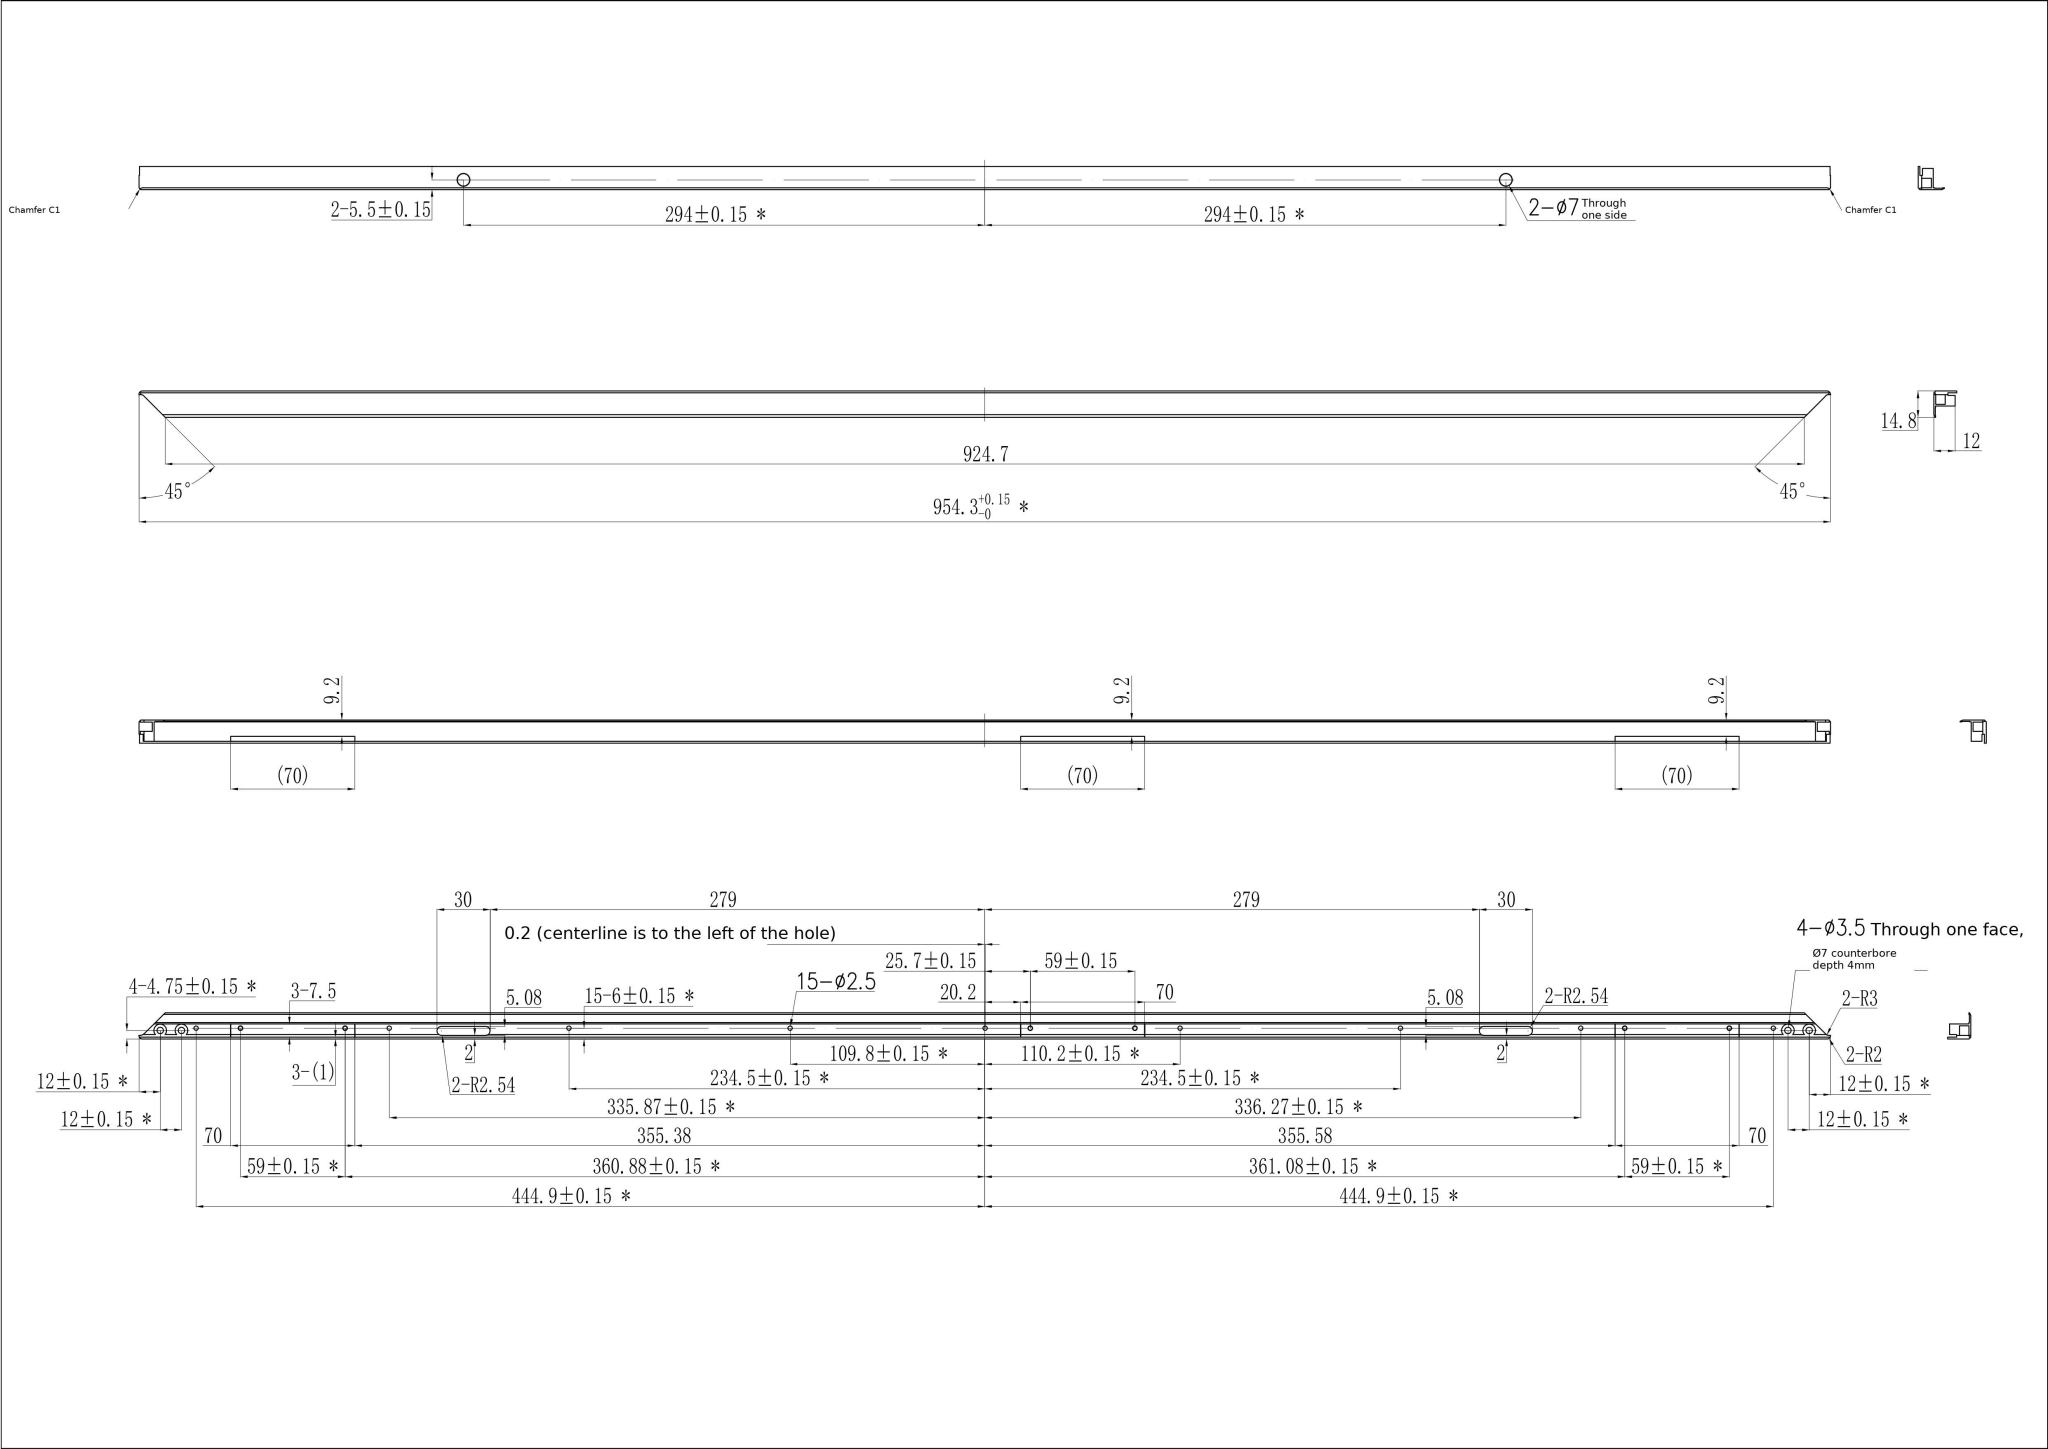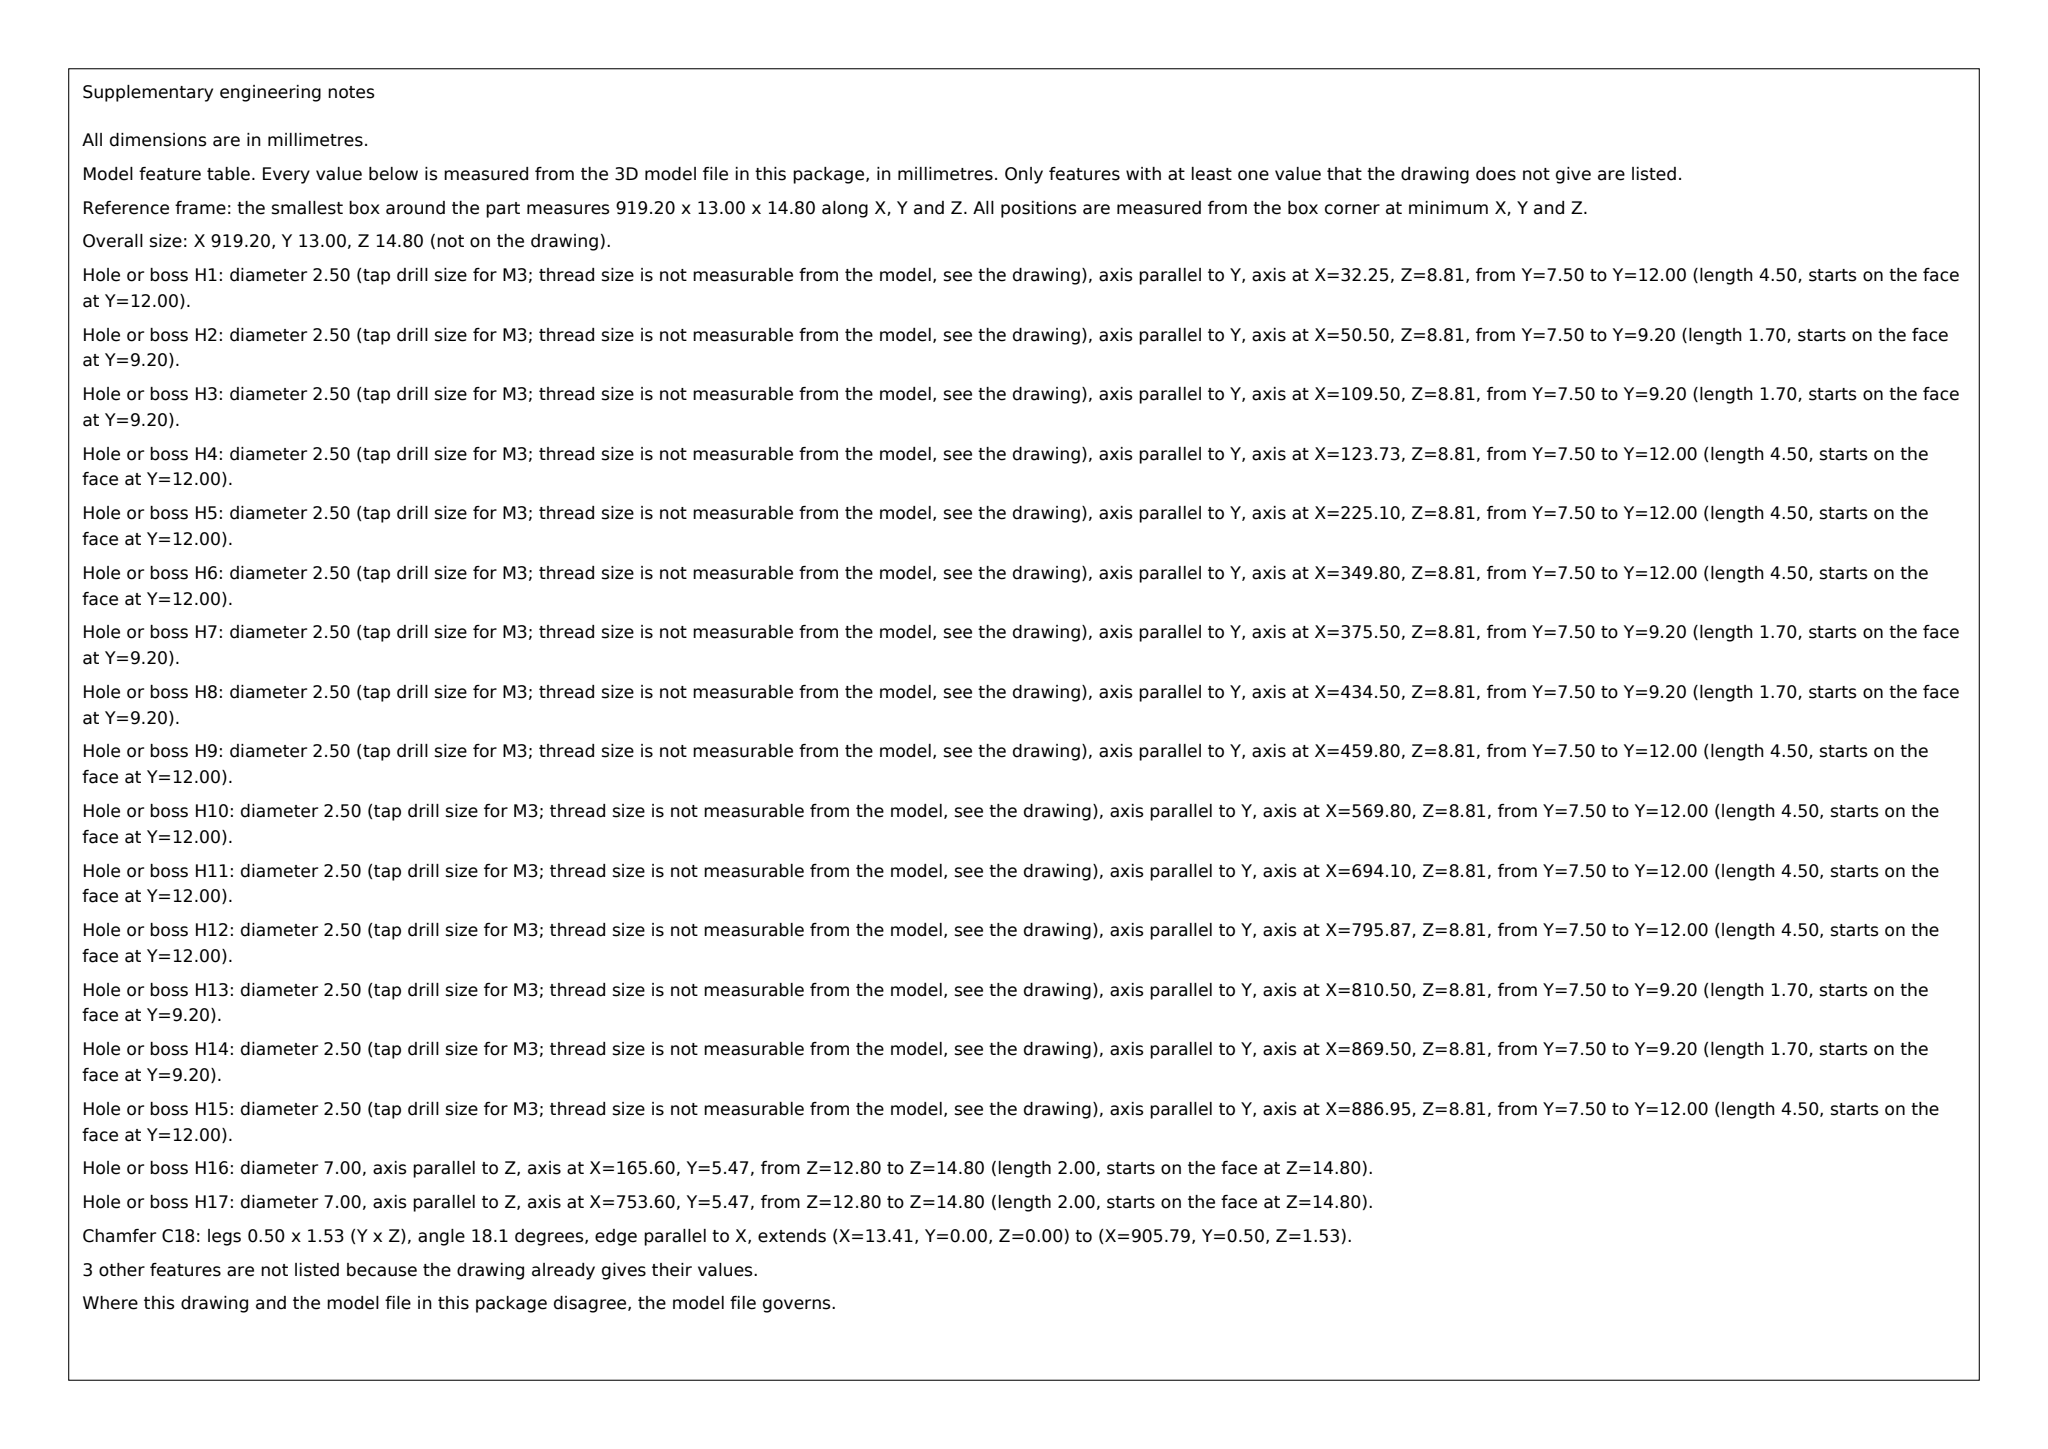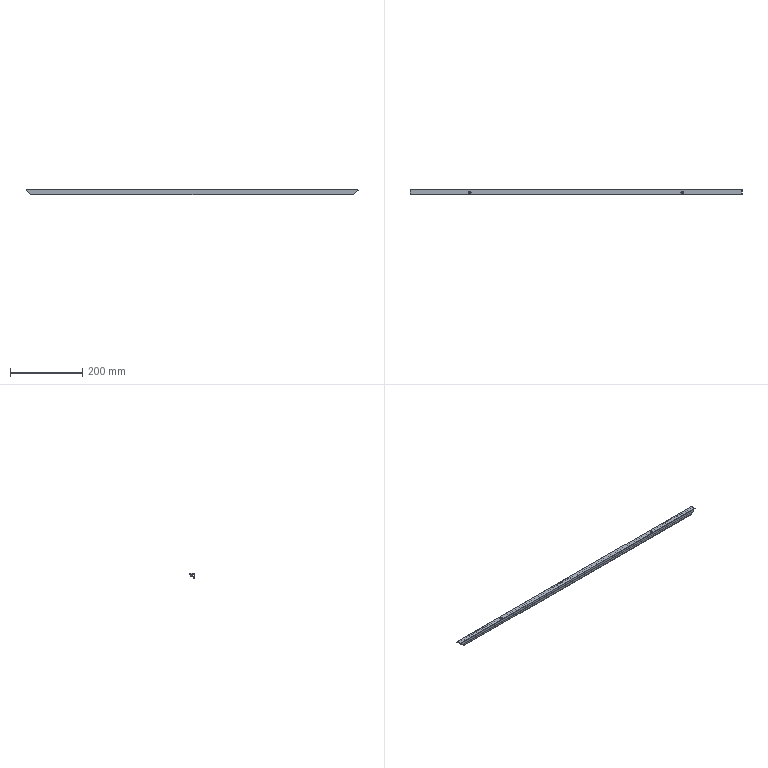Part | SolidWorks | mm | 1 solid | 104 faces | box 919.2 x 13 x 14.8 mm | volume 62018 mm3 | plane 68 | cylinder 36 | commonest cylinder face diameters 2.5 x30 7 x4 4 x2